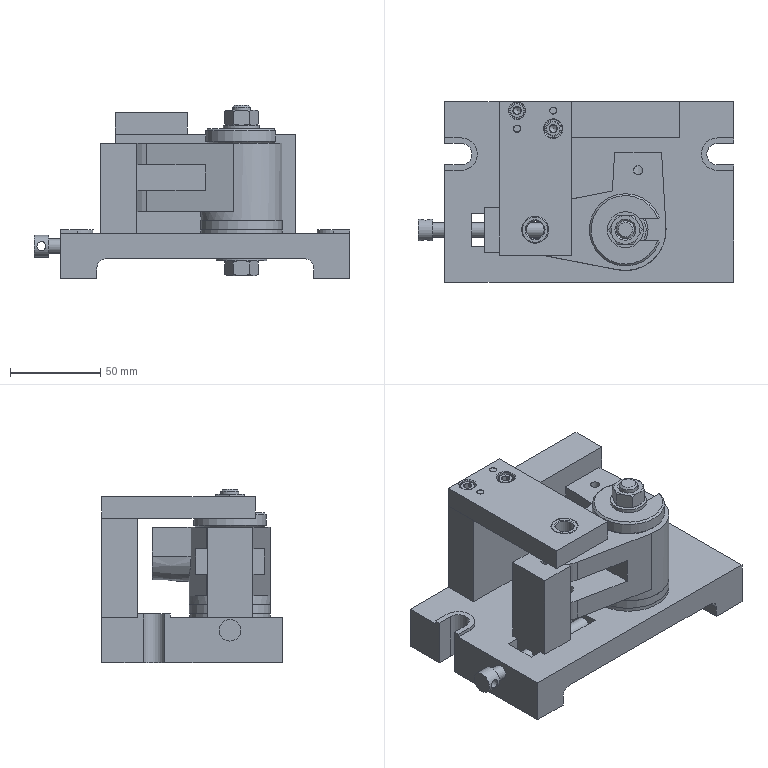Assembly | NX | mm | 16 component files | 16 solids | 274 faces | box 174.76 x 100 x 96 mm | volume 542380 mm3 | plane 142 | cone 70 | cylinder 57 | torus 4 | spline 1 | commonest cylinder face diameters 10 x12 4 x6 12 x5 25 x4 4.826 x4 8 x4 45 x3 18 x2
Bill of materials:
unnamed part 1 | 1 |  | Stepped round shaft: a long thin pin on one side, a larger cylindrical hub in the middle with a thin disc flange around it, and a short thin pin on the other side.
unnamed part 2 | 1 |  | Long rectangular block with a V-groove down its length. The bottom of the V has a narrow rectangular slot. One end narrows to a tab with a round through-hole across it.
unnamed part 3 | 1 |  | Hollow cylindrical sleeve: a thick-walled tube with a plain through-bore and chamfered outer edges at both ends.
unnamed part 4 | 1 |  | Flat circular ring (washer-like annulus) with a central through-hole and square, unchamfered edges.
GB-T70.1-2000,M5x16 | 2 |  | ÄÚÁù½ÇÔ²ÖùÍ·ÂÝ¶¤
unnamed part 5 | 1 |  | Lever or arm-like bracket with a cylindrical hub. The hub has a large bore with a keyway notch. A tapered arm with a round end and a hole is split by a slot into two forks. A second short arm has a small hole, and the side of the hub has a cross-hole.
unnamed part 6 | 2 |  | Plain solid cylindrical pin with chamfered edges at both ends.
unnamed part 7 | 1 |  | C-shaped slotted washer: a flat disc with a slot that runs from the edge to the centre, ending in a rounded inner end, with chamfered edges.
unnamed part 8 | 1 |  | Headed pin: a long cylindrical shank with a chamfered tip and a larger cylindrical head. A small hole runs across the head.
unnamed part 9 | 1 |  | Flat rectangular plate. One large round through-hole sits near one end. Near the other end are two medium holes with counterbore rings and two small plain holes.
GB-T6170_F-2000,M10x1.5 | 2 |  | Hexagonal nut-like body: a six-sided prism with a central through-bore and chamfered corners at both ends.
unnamed part 10 | 1 |  | Thin flat washer-like disc with a large outer diameter compared with its central hole.
unnamed part 11 | 1 |  | Rectangular base plate with an upright rectangular wall block along one edge. The base has U-shaped notches on both ends, a rectangular through-slot, a round through-hole with a spotface or counterbore ring, and an underside relief channel. The top of the upright has four small holes.
Mates:
1. fix | fixture_body 1 component
2. touch align | mandrel 1 face | fixture_body 1 face
3. touch align | mandrel 1 face | fixture_body 1 face
4. touch align | drill_jig 1 face | fixture_body 1 face
5. touch align | drill_jig 1 face | fixture_body 1 face
6. touch align | handle_base 1 face | mandrel 1 face
7. touch align | handle_base 1 face | drill_jig 1 face
8. touch align | handle_base 1 face | mandrel 1 face
9. touch align | split_washer 1 face | handle_base 1 face
10. concentric | cyl_pin 2 edge | drill_jig 1 edge
11. concentric | cyl_pin 1 edge | drill_jig 1 edge
12. touch align | bushing 1 face | drill_jig 1 face
13. concentric | bushing 1 edge | drill_jig 1 arc
14. touch align | screw 2 face | drill_jig 1 face
15. touch align | screw 2 face | drill_jig 1 face
16. touch align | screw 1 face | drill_jig 1 face
17. touch align | screw 1 face | drill_jig 1 face
18. touch align | flat_washer 1 face | split_washer 1 face
19. touch align | flat_washer 1 face | mandrel 1 face
20. touch align | nut 2 face | flat_washer 1 face
21. touch align | washer 1 face | fixture_body 1 face
22. touch align | washer 1 face | mandrel 1 face
23. touch align | nut 1 face | washer 1 face
24. touch align | nut 1 face | mandrel 1 face
25. center | v_block 1 | v_block 1 | fixture_body 1 face | fixture_body 1 face
26. touch align | v_block 1 | fixture_body 1 face
27. touch align | torque_shaft 1 face | fixture_body 1 face
28. touch align | torque_shaft 1 edge | fixture_body 1 face
29. touch align | v_block 1 face | handle_base 1 face
30. touch align | v_block 1 face | handle_base 1 face